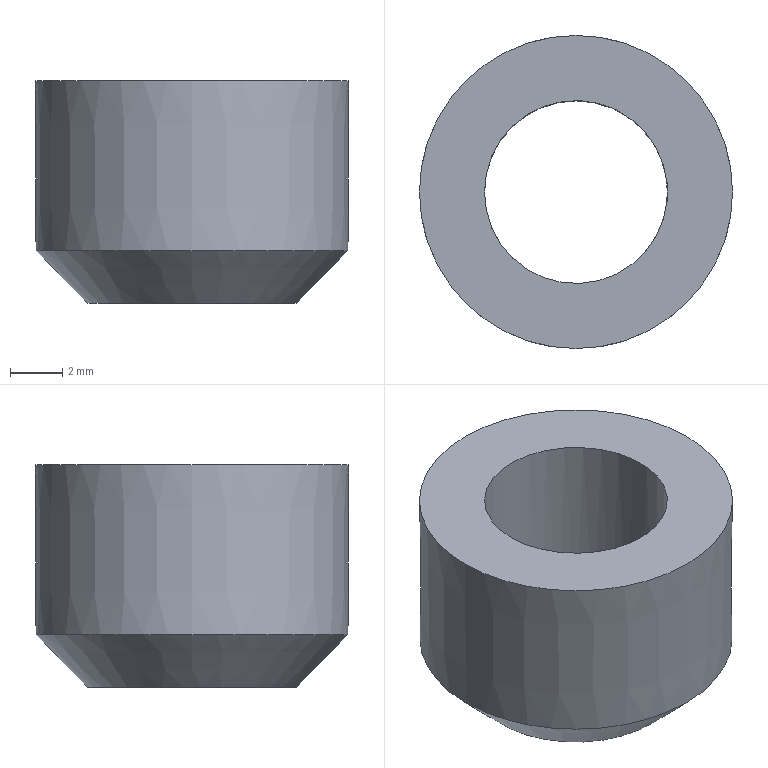Component | NX | PACKING | 1 solid | 5 faces | box 11.98 x 11.98 x 8.5 mm | volume 561 mm3 | plane 2 | cone 2 | cylinder 1 | commonest cylinder face diameters 7 x1
STEP:
#1=CARTESIAN_POINT('',(0.,0.,0.));
#2=DIRECTION('',(0.,0.,1.));
#3=DIRECTION('',(1.,0.,0.));
#4=AXIS2_PLACEMENT_3D('',#1,#2,#3);
#5=CARTESIAN_POINT('',(3.5,0.,63.5));
#6=VERTEX_POINT('',#5);
#7=CARTESIAN_POINT('',(-3.5,0.,63.5));
#8=VERTEX_POINT('',#7);
#9=CARTESIAN_POINT('',(0.,0.,63.5));
#10=DIRECTION('',(0.,0.,1.));
#11=DIRECTION('',(1.,0.,0.));
#12=AXIS2_PLACEMENT_3D('',#9,#10,#11);
#13=CIRCLE('',#12,3.5);
#14=CARTESIAN_POINT('',(0.,0.,63.5));
#15=DIRECTION('',(0.,0.,1.));
#16=DIRECTION('',(1.,0.,0.));
#17=AXIS2_PLACEMENT_3D('',#14,#15,#16);
#18=PLANE('',#17);
#19=CARTESIAN_POINT('',(0.,0.));
#20=DIRECTION('',(1.,0.));
#21=AXIS2_PLACEMENT_2D('',#19,#20);
#22=CIRCLE('',#21,3.5);
#23=(GEOMETRIC_REPRESENTATION_CONTEXT(2)PARAMETRIC_REPRESENTATION_CONTEXT()REPRESENTATION_CONTEXT('',''));
#24=DEFINITIONAL_REPRESENTATION('',(#22),#23);
#25=PCURVE('',#18,#24);
#26=CARTESIAN_POINT('',(0.,0.,72.));
#27=DIRECTION('',(0.,0.,-1.));
#28=DIRECTION('',(-1.,0.,0.));
#29=AXIS2_PLACEMENT_3D('',#26,#27,#28);
#30=CYLINDRICAL_SURFACE('',#29,3.5);
#31=CARTESIAN_POINT('',(3.142,8.5));
#32=DIRECTION('',(-1.,0.));
#33=VECTOR('',#32,1.);
#34=LINE('',#31,#33);
#35=(GEOMETRIC_REPRESENTATION_CONTEXT(2)PARAMETRIC_REPRESENTATION_CONTEXT()REPRESENTATION_CONTEXT('',''));
#36=DEFINITIONAL_REPRESENTATION('',(#34),#35);
#37=PCURVE('',#30,#36);
#38=SURFACE_CURVE('',#13,(#25,#37),.PCURVE_S1.);
#39=EDGE_CURVE('',#6,#8,#38,.T.);
#40=ORIENTED_EDGE('',*,*,#39,.T.);
#41=CARTESIAN_POINT('',(0.,0.,63.5));
#42=DIRECTION('',(0.,0.,1.));
#43=DIRECTION('',(1.,0.,0.));
#44=AXIS2_PLACEMENT_3D('',#41,#42,#43);
#45=CIRCLE('',#44,3.5);
#46=CARTESIAN_POINT('',(0.,0.));
#47=DIRECTION('',(1.,0.));
#48=AXIS2_PLACEMENT_2D('',#46,#47);
#49=CIRCLE('',#48,3.5);
#50=(GEOMETRIC_REPRESENTATION_CONTEXT(2)PARAMETRIC_REPRESENTATION_CONTEXT()REPRESENTATION_CONTEXT('',''));
#51=DEFINITIONAL_REPRESENTATION('',(#49),#50);
#52=PCURVE('',#18,#51);
#53=CARTESIAN_POINT('',(9.425,8.5));
#54=DIRECTION('',(-1.,0.));
#55=VECTOR('',#54,1.);
#56=LINE('',#53,#55);
#57=(GEOMETRIC_REPRESENTATION_CONTEXT(2)PARAMETRIC_REPRESENTATION_CONTEXT()REPRESENTATION_CONTEXT('',''));
#58=DEFINITIONAL_REPRESENTATION('',(#56),#57);
#59=PCURVE('',#30,#58);
#60=SURFACE_CURVE('',#45,(#52,#59),.PCURVE_S1.);
#61=EDGE_CURVE('',#8,#6,#60,.T.);
#62=ORIENTED_EDGE('',*,*,#61,.T.);
#63=EDGE_LOOP('',(#40,#62));
#64=FACE_BOUND('',#63,.T.);
#65=CARTESIAN_POINT('',(4.,0.,63.5));
#66=VERTEX_POINT('',#65);
#67=CARTESIAN_POINT('',(0.,0.,63.5));
#68=DIRECTION('',(0.,0.,1.));
#69=DIRECTION('',(1.,0.,0.));
#70=AXIS2_PLACEMENT_3D('',#67,#68,#69);
#71=CIRCLE('',#70,4.);
#72=CARTESIAN_POINT('',(0.,0.));
#73=DIRECTION('',(1.,0.));
#74=AXIS2_PLACEMENT_2D('',#72,#73);
#75=CIRCLE('',#74,4.);
#76=(GEOMETRIC_REPRESENTATION_CONTEXT(2)PARAMETRIC_REPRESENTATION_CONTEXT()REPRESENTATION_CONTEXT('',''));
#77=DEFINITIONAL_REPRESENTATION('',(#75),#76);
#78=PCURVE('',#18,#77);
#79=CARTESIAN_POINT('',(0.,0.,63.5));
#80=DIRECTION('',(0.,0.,1.));
#81=DIRECTION('',(1.,0.,0.));
#82=AXIS2_PLACEMENT_3D('',#79,#80,#81);
#83=CONICAL_SURFACE('',#82,4.,0.7771);
#84=CARTESIAN_POINT('',(0.,0.));
#85=DIRECTION('',(1.,0.));
#86=VECTOR('',#85,1.);
#87=LINE('',#84,#86);
#88=(GEOMETRIC_REPRESENTATION_CONTEXT(2)PARAMETRIC_REPRESENTATION_CONTEXT()REPRESENTATION_CONTEXT('',''));
#89=DEFINITIONAL_REPRESENTATION('',(#87),#88);
#90=PCURVE('',#83,#89);
#91=SURFACE_CURVE('',#71,(#78,#90),.PCURVE_S1.);
#92=EDGE_CURVE('',#66,#66,#91,.T.);
#93=ORIENTED_EDGE('',*,*,#92,.F.);
#94=EDGE_LOOP('',(#93));
#95=FACE_BOUND('',#94,.T.);
#96=ADVANCED_FACE('',(#64,#95),#18,.F.);
#97=CARTESIAN_POINT('',(5.967,0.,65.5));
#98=VERTEX_POINT('',#97);
#99=CARTESIAN_POINT('',(0.,0.,65.5));
#100=DIRECTION('',(0.,0.,1.));
#101=DIRECTION('',(1.,0.,0.));
#102=AXIS2_PLACEMENT_3D('',#99,#100,#101);
#103=CIRCLE('',#102,5.967);
#104=CARTESIAN_POINT('',(0.,2.));
#105=DIRECTION('',(1.,0.));
#106=VECTOR('',#105,1.);
#107=LINE('',#104,#106);
#108=(GEOMETRIC_REPRESENTATION_CONTEXT(2)PARAMETRIC_REPRESENTATION_CONTEXT()REPRESENTATION_CONTEXT('',''));
#109=DEFINITIONAL_REPRESENTATION('',(#107),#108);
#110=PCURVE('',#83,#109);
#111=CARTESIAN_POINT('',(0.,0.,65.5));
#112=DIRECTION('',(0.,0.,1.));
#113=DIRECTION('',(1.,0.,0.));
#114=AXIS2_PLACEMENT_3D('',#111,#112,#113);
#115=CONICAL_SURFACE('',#114,5.967,0.003469);
#116=CARTESIAN_POINT('',(0.,0.));
#117=DIRECTION('',(1.,0.));
#118=VECTOR('',#117,1.);
#119=LINE('',#116,#118);
#120=(GEOMETRIC_REPRESENTATION_CONTEXT(2)PARAMETRIC_REPRESENTATION_CONTEXT()REPRESENTATION_CONTEXT('',''));
#121=DEFINITIONAL_REPRESENTATION('',(#119),#120);
#122=PCURVE('',#115,#121);
#123=SURFACE_CURVE('',#103,(#110,#122),.PCURVE_S1.);
#124=EDGE_CURVE('',#98,#98,#123,.T.);
#125=ORIENTED_EDGE('',*,*,#124,.F.);
#126=CARTESIAN_POINT('',(4.,-0.,63.5));
#127=CARTESIAN_POINT('',(5.967,-0.,65.5));
#128=B_SPLINE_CURVE_WITH_KNOTS('',1,(#126,#127),.UNSPECIFIED.,.F.,.F.,(2,2),(0.,2.805),.PIECEWISE_BEZIER_KNOTS.);
#129=CARTESIAN_POINT('',(0.,0.));
#130=DIRECTION('',(0.,1.));
#131=VECTOR('',#130,1.);
#132=LINE('',#129,#131);
#133=(GEOMETRIC_REPRESENTATION_CONTEXT(2)PARAMETRIC_REPRESENTATION_CONTEXT()REPRESENTATION_CONTEXT('',''));
#134=DEFINITIONAL_REPRESENTATION('',(#132),#133);
#135=PCURVE('',#83,#134);
#136=CARTESIAN_POINT('',(6.283,0.));
#137=DIRECTION('',(0.,1.));
#138=VECTOR('',#137,1.);
#139=LINE('',#136,#138);
#140=(GEOMETRIC_REPRESENTATION_CONTEXT(2)PARAMETRIC_REPRESENTATION_CONTEXT()REPRESENTATION_CONTEXT('',''));
#141=DEFINITIONAL_REPRESENTATION('',(#139),#140);
#142=PCURVE('',#83,#141);
#143=SEAM_CURVE('',#128,(#135,#142),.PCURVE_S1.);
#144=EDGE_CURVE('',#66,#98,#143,.T.);
#145=ORIENTED_EDGE('',*,*,#144,.F.);
#146=ORIENTED_EDGE('',*,*,#92,.T.);
#147=ORIENTED_EDGE('',*,*,#144,.T.);
#148=EDGE_LOOP('',(#125,#145,#146,#147));
#149=FACE_BOUND('',#148,.T.);
#150=ADVANCED_FACE('',(#149),#83,.T.);
#151=CARTESIAN_POINT('',(5.99,0.,72.));
#152=VERTEX_POINT('',#151);
#153=CARTESIAN_POINT('',(-5.99,0.,72.));
#154=VERTEX_POINT('',#153);
#155=CARTESIAN_POINT('',(0.,0.,72.));
#156=DIRECTION('',(0.,0.,1.));
#157=DIRECTION('',(-1.,0.,0.));
#158=AXIS2_PLACEMENT_3D('',#155,#156,#157);
#159=CIRCLE('',#158,5.99);
#160=CARTESIAN_POINT('',(-3.142,6.5));
#161=DIRECTION('',(1.,0.));
#162=VECTOR('',#161,1.);
#163=LINE('',#160,#162);
#164=(GEOMETRIC_REPRESENTATION_CONTEXT(2)PARAMETRIC_REPRESENTATION_CONTEXT()REPRESENTATION_CONTEXT('',''));
#165=DEFINITIONAL_REPRESENTATION('',(#163),#164);
#166=PCURVE('',#115,#165);
#167=CARTESIAN_POINT('',(0.,5.981,72.));
#168=DIRECTION('',(0.,0.,-1.));
#169=DIRECTION('',(-1.,0.,0.));
#170=AXIS2_PLACEMENT_3D('',#167,#168,#169);
#171=PLANE('',#170);
#172=CARTESIAN_POINT('',(5.99,-5.981));
#173=CARTESIAN_POINT('',(5.99,-16.356));
#174=CARTESIAN_POINT('',(-2.995,-11.168));
#175=CARTESIAN_POINT('',(-11.98,-5.981));
#176=CARTESIAN_POINT('',(-2.995,-0.7938));
#177=CARTESIAN_POINT('',(5.99,4.393));
#178=CARTESIAN_POINT('',(5.99,-5.981));
#179=(BOUNDED_CURVE()B_SPLINE_CURVE(2,(#172,#173,#174,#175,#176,#177,#178),.UNSPECIFIED.,.T.,.F.)B_SPLINE_CURVE_WITH_KNOTS((1,2,2,2,2,1),(-2.094,0.,2.094,4.189,6.283,8.378),.UNSPECIFIED.)CURVE()GEOMETRIC_REPRESENTATION_ITEM()RATIONAL_B_SPLINE_CURVE((1.,0.5,1.,0.5,1.,0.5,1.))REPRESENTATION_ITEM(''));
#180=(GEOMETRIC_REPRESENTATION_CONTEXT(2)PARAMETRIC_REPRESENTATION_CONTEXT()REPRESENTATION_CONTEXT('',''));
#181=DEFINITIONAL_REPRESENTATION('',(#179),#180);
#182=PCURVE('',#171,#181);
#183=SURFACE_CURVE('',#159,(#166,#182),.PCURVE_S1.);
#184=EDGE_CURVE('',#152,#154,#183,.T.);
#185=ORIENTED_EDGE('',*,*,#184,.F.);
#186=CARTESIAN_POINT('',(5.967,-0.,65.5));
#187=CARTESIAN_POINT('',(5.99,-0.,72.));
#188=B_SPLINE_CURVE_WITH_KNOTS('',1,(#186,#187),.UNSPECIFIED.,.F.,.F.,(2,2),(0.,6.5),.PIECEWISE_BEZIER_KNOTS.);
#189=CARTESIAN_POINT('',(0.,0.));
#190=DIRECTION('',(0.,1.));
#191=VECTOR('',#190,1.);
#192=LINE('',#189,#191);
#193=(GEOMETRIC_REPRESENTATION_CONTEXT(2)PARAMETRIC_REPRESENTATION_CONTEXT()REPRESENTATION_CONTEXT('',''));
#194=DEFINITIONAL_REPRESENTATION('',(#192),#193);
#195=PCURVE('',#115,#194);
#196=CARTESIAN_POINT('',(6.283,0.));
#197=DIRECTION('',(0.,1.));
#198=VECTOR('',#197,1.);
#199=LINE('',#196,#198);
#200=(GEOMETRIC_REPRESENTATION_CONTEXT(2)PARAMETRIC_REPRESENTATION_CONTEXT()REPRESENTATION_CONTEXT('',''));
#201=DEFINITIONAL_REPRESENTATION('',(#199),#200);
#202=PCURVE('',#115,#201);
#203=SEAM_CURVE('',#188,(#195,#202),.PCURVE_S1.);
#204=EDGE_CURVE('',#98,#152,#203,.T.);
#205=ORIENTED_EDGE('',*,*,#204,.F.);
#206=ORIENTED_EDGE('',*,*,#124,.T.);
#207=ORIENTED_EDGE('',*,*,#204,.T.);
#208=CARTESIAN_POINT('',(0.,0.,72.));
#209=DIRECTION('',(0.,0.,1.));
#210=DIRECTION('',(-1.,0.,0.));
#211=AXIS2_PLACEMENT_3D('',#208,#209,#210);
#212=CIRCLE('',#211,5.99);
#213=CARTESIAN_POINT('',(3.142,6.5));
#214=DIRECTION('',(1.,0.));
#215=VECTOR('',#214,1.);
#216=LINE('',#213,#215);
#217=(GEOMETRIC_REPRESENTATION_CONTEXT(2)PARAMETRIC_REPRESENTATION_CONTEXT()REPRESENTATION_CONTEXT('',''));
#218=DEFINITIONAL_REPRESENTATION('',(#216),#217);
#219=PCURVE('',#115,#218);
#220=CARTESIAN_POINT('',(5.99,-5.981));
#221=CARTESIAN_POINT('',(5.99,-16.356));
#222=CARTESIAN_POINT('',(-2.995,-11.168));
#223=CARTESIAN_POINT('',(-11.98,-5.981));
#224=CARTESIAN_POINT('',(-2.995,-0.7938));
#225=CARTESIAN_POINT('',(5.99,4.393));
#226=CARTESIAN_POINT('',(5.99,-5.981));
#227=(BOUNDED_CURVE()B_SPLINE_CURVE(2,(#220,#221,#222,#223,#224,#225,#226),.UNSPECIFIED.,.T.,.F.)B_SPLINE_CURVE_WITH_KNOTS((1,2,2,2,2,1),(-2.094,0.,2.094,4.189,6.283,8.378),.UNSPECIFIED.)CURVE()GEOMETRIC_REPRESENTATION_ITEM()RATIONAL_B_SPLINE_CURVE((1.,0.5,1.,0.5,1.,0.5,1.))REPRESENTATION_ITEM(''));
#228=(GEOMETRIC_REPRESENTATION_CONTEXT(2)PARAMETRIC_REPRESENTATION_CONTEXT()REPRESENTATION_CONTEXT('',''));
#229=DEFINITIONAL_REPRESENTATION('',(#227),#228);
#230=PCURVE('',#171,#229);
#231=SURFACE_CURVE('',#212,(#219,#230),.PCURVE_S1.);
#232=EDGE_CURVE('',#154,#152,#231,.T.);
#233=ORIENTED_EDGE('',*,*,#232,.F.);
#234=EDGE_LOOP('',(#185,#205,#206,#207,#233));
#235=FACE_BOUND('',#234,.T.);
#236=ADVANCED_FACE('',(#235),#115,.T.);
#237=CARTESIAN_POINT('',(-3.5,0.,72.));
#238=VERTEX_POINT('',#237);
#239=CARTESIAN_POINT('',(0.,0.,72.));
#240=DIRECTION('',(0.,0.,-1.));
#241=DIRECTION('',(-1.,0.,0.));
#242=AXIS2_PLACEMENT_3D('',#239,#240,#241);
#243=CIRCLE('',#242,3.5);
#244=CARTESIAN_POINT('',(0.,-5.981));
#245=DIRECTION('',(1.,0.));
#246=AXIS2_PLACEMENT_2D('',#244,#245);
#247=CIRCLE('',#246,3.5);
#248=(GEOMETRIC_REPRESENTATION_CONTEXT(2)PARAMETRIC_REPRESENTATION_CONTEXT()REPRESENTATION_CONTEXT('',''));
#249=DEFINITIONAL_REPRESENTATION('',(#247),#248);
#250=PCURVE('',#171,#249);
#251=CARTESIAN_POINT('',(0.,0.));
#252=DIRECTION('',(1.,0.));
#253=VECTOR('',#252,1.);
#254=LINE('',#251,#253);
#255=(GEOMETRIC_REPRESENTATION_CONTEXT(2)PARAMETRIC_REPRESENTATION_CONTEXT()REPRESENTATION_CONTEXT('',''));
#256=DEFINITIONAL_REPRESENTATION('',(#254),#255);
#257=PCURVE('',#30,#256);
#258=SURFACE_CURVE('',#243,(#250,#257),.PCURVE_S1.);
#259=EDGE_CURVE('',#238,#238,#258,.T.);
#260=ORIENTED_EDGE('',*,*,#259,.T.);
#261=EDGE_LOOP('',(#260));
#262=FACE_BOUND('',#261,.T.);
#263=ORIENTED_EDGE('',*,*,#232,.T.);
#264=ORIENTED_EDGE('',*,*,#184,.T.);
#265=EDGE_LOOP('',(#263,#264));
#266=FACE_BOUND('',#265,.T.);
#267=ADVANCED_FACE('',(#262,#266),#171,.F.);
#268=ORIENTED_EDGE('',*,*,#259,.T.);
#269=CARTESIAN_POINT('',(-3.5,0.,72.));
#270=CARTESIAN_POINT('',(-3.5,0.,63.5));
#271=B_SPLINE_CURVE_WITH_KNOTS('',1,(#269,#270),.UNSPECIFIED.,.F.,.F.,(2,2),(0.,8.5),.PIECEWISE_BEZIER_KNOTS.);
#272=CARTESIAN_POINT('',(6.283,0.));
#273=DIRECTION('',(0.,1.));
#274=VECTOR('',#273,1.);
#275=LINE('',#272,#274);
#276=(GEOMETRIC_REPRESENTATION_CONTEXT(2)PARAMETRIC_REPRESENTATION_CONTEXT()REPRESENTATION_CONTEXT('',''));
#277=DEFINITIONAL_REPRESENTATION('',(#275),#276);
#278=PCURVE('',#30,#277);
#279=CARTESIAN_POINT('',(0.,0.));
#280=DIRECTION('',(0.,1.));
#281=VECTOR('',#280,1.);
#282=LINE('',#279,#281);
#283=(GEOMETRIC_REPRESENTATION_CONTEXT(2)PARAMETRIC_REPRESENTATION_CONTEXT()REPRESENTATION_CONTEXT('',''));
#284=DEFINITIONAL_REPRESENTATION('',(#282),#283);
#285=PCURVE('',#30,#284);
#286=SEAM_CURVE('',#271,(#278,#285),.PCURVE_S1.);
#287=EDGE_CURVE('',#238,#8,#286,.T.);
#288=ORIENTED_EDGE('',*,*,#287,.T.);
#289=ORIENTED_EDGE('',*,*,#61,.T.);
#290=ORIENTED_EDGE('',*,*,#39,.T.);
#291=ORIENTED_EDGE('',*,*,#287,.F.);
#292=EDGE_LOOP('',(#268,#288,#289,#290,#291));
#293=FACE_BOUND('',#292,.F.);
#294=ADVANCED_FACE('',(#293),#30,.F.);
#295=CLOSED_SHELL('',(#96,#150,#236,#267,#294));
#296=MANIFOLD_SOLID_BREP('',#295);
#297=(LENGTH_UNIT()NAMED_UNIT(*)SI_UNIT(.MILLI.,.METRE.));
#298=UNCERTAINTY_MEASURE_WITH_UNIT(LENGTH_MEASURE(0.000005),#297,'','');
#299=(NAMED_UNIT(*)PLANE_ANGLE_UNIT()SI_UNIT($,.RADIAN.));
#300=(NAMED_UNIT(*)SI_UNIT($,.STERADIAN.)SOLID_ANGLE_UNIT());
#301=(GEOMETRIC_REPRESENTATION_CONTEXT(3)GLOBAL_UNCERTAINTY_ASSIGNED_CONTEXT((#298))GLOBAL_UNIT_ASSIGNED_CONTEXT((#297,#299,#300))REPRESENTATION_CONTEXT('',''));
#302=ADVANCED_BREP_SHAPE_REPRESENTATION('',(#4,#296),#301);